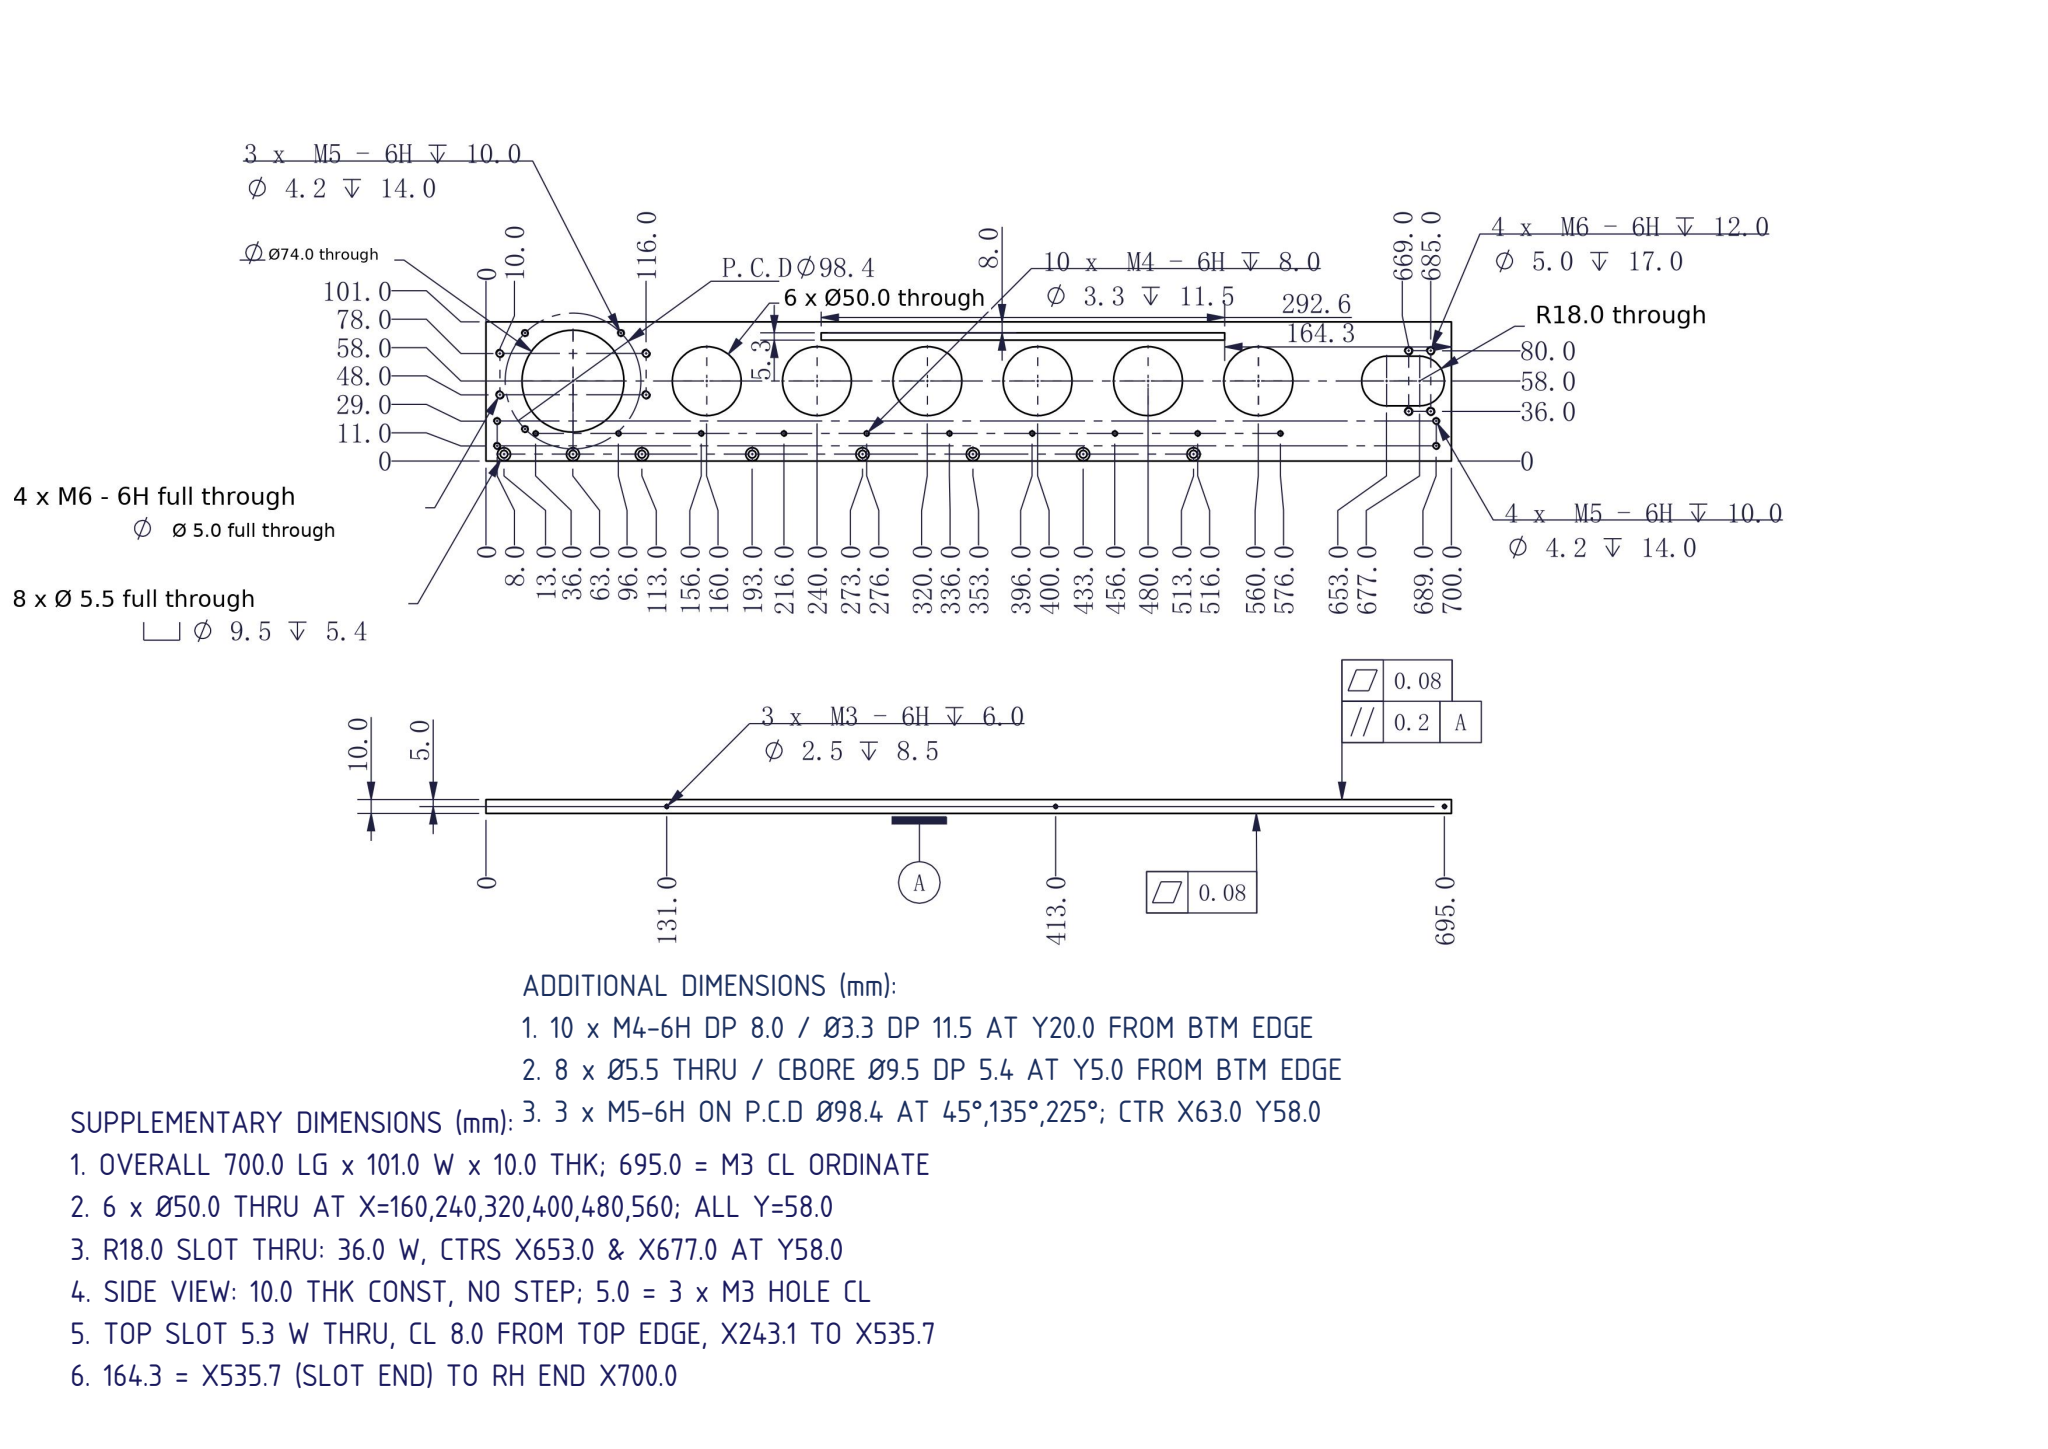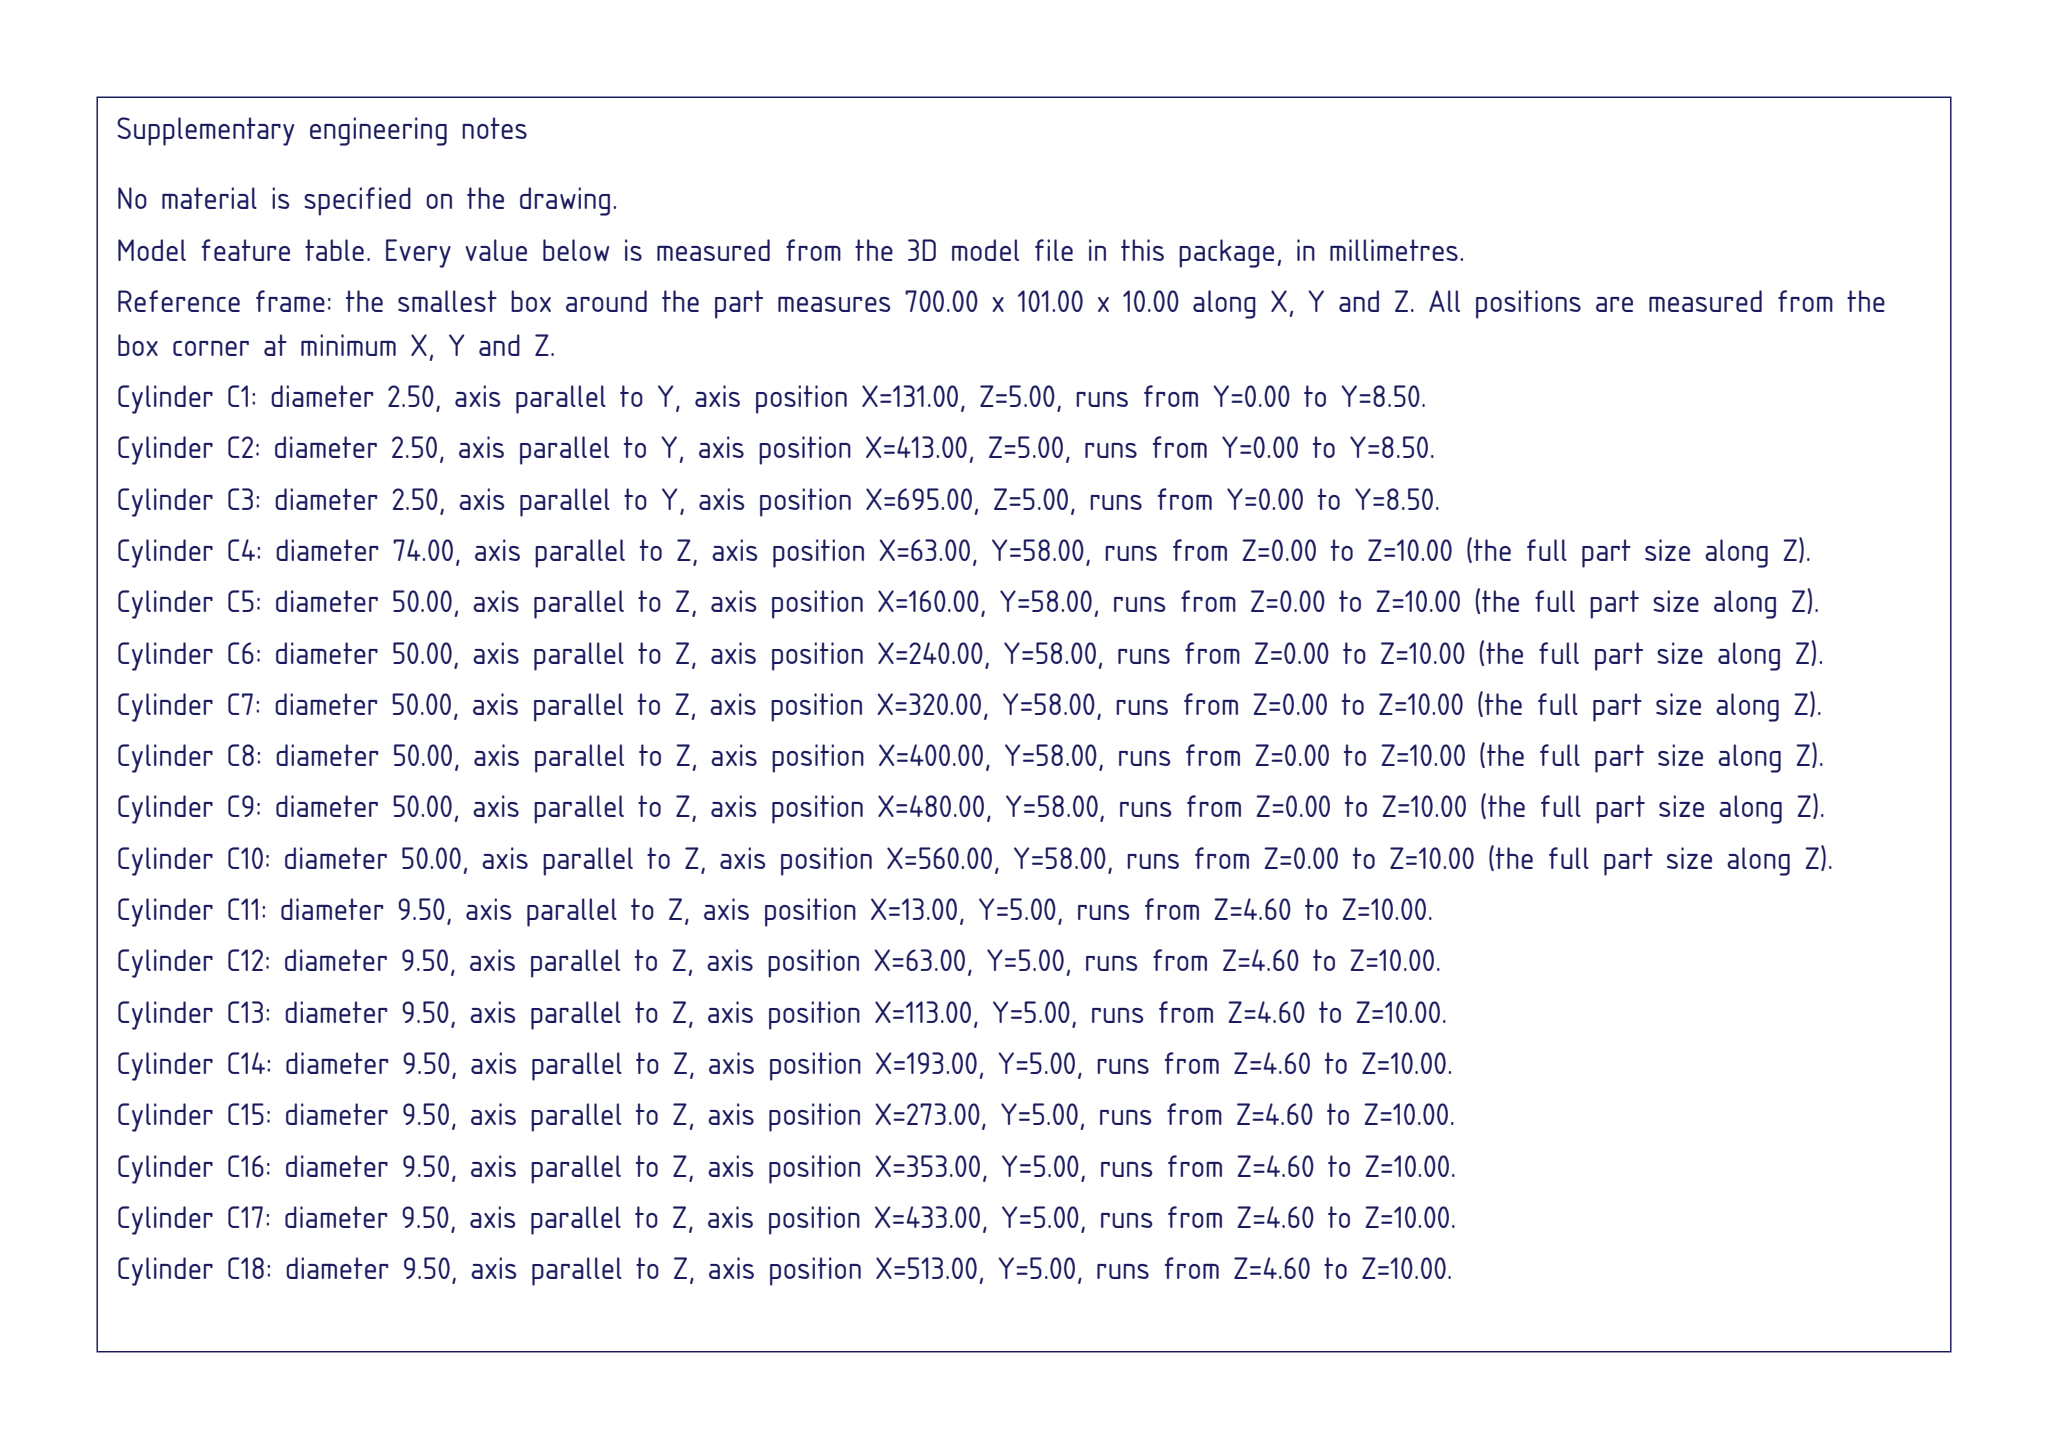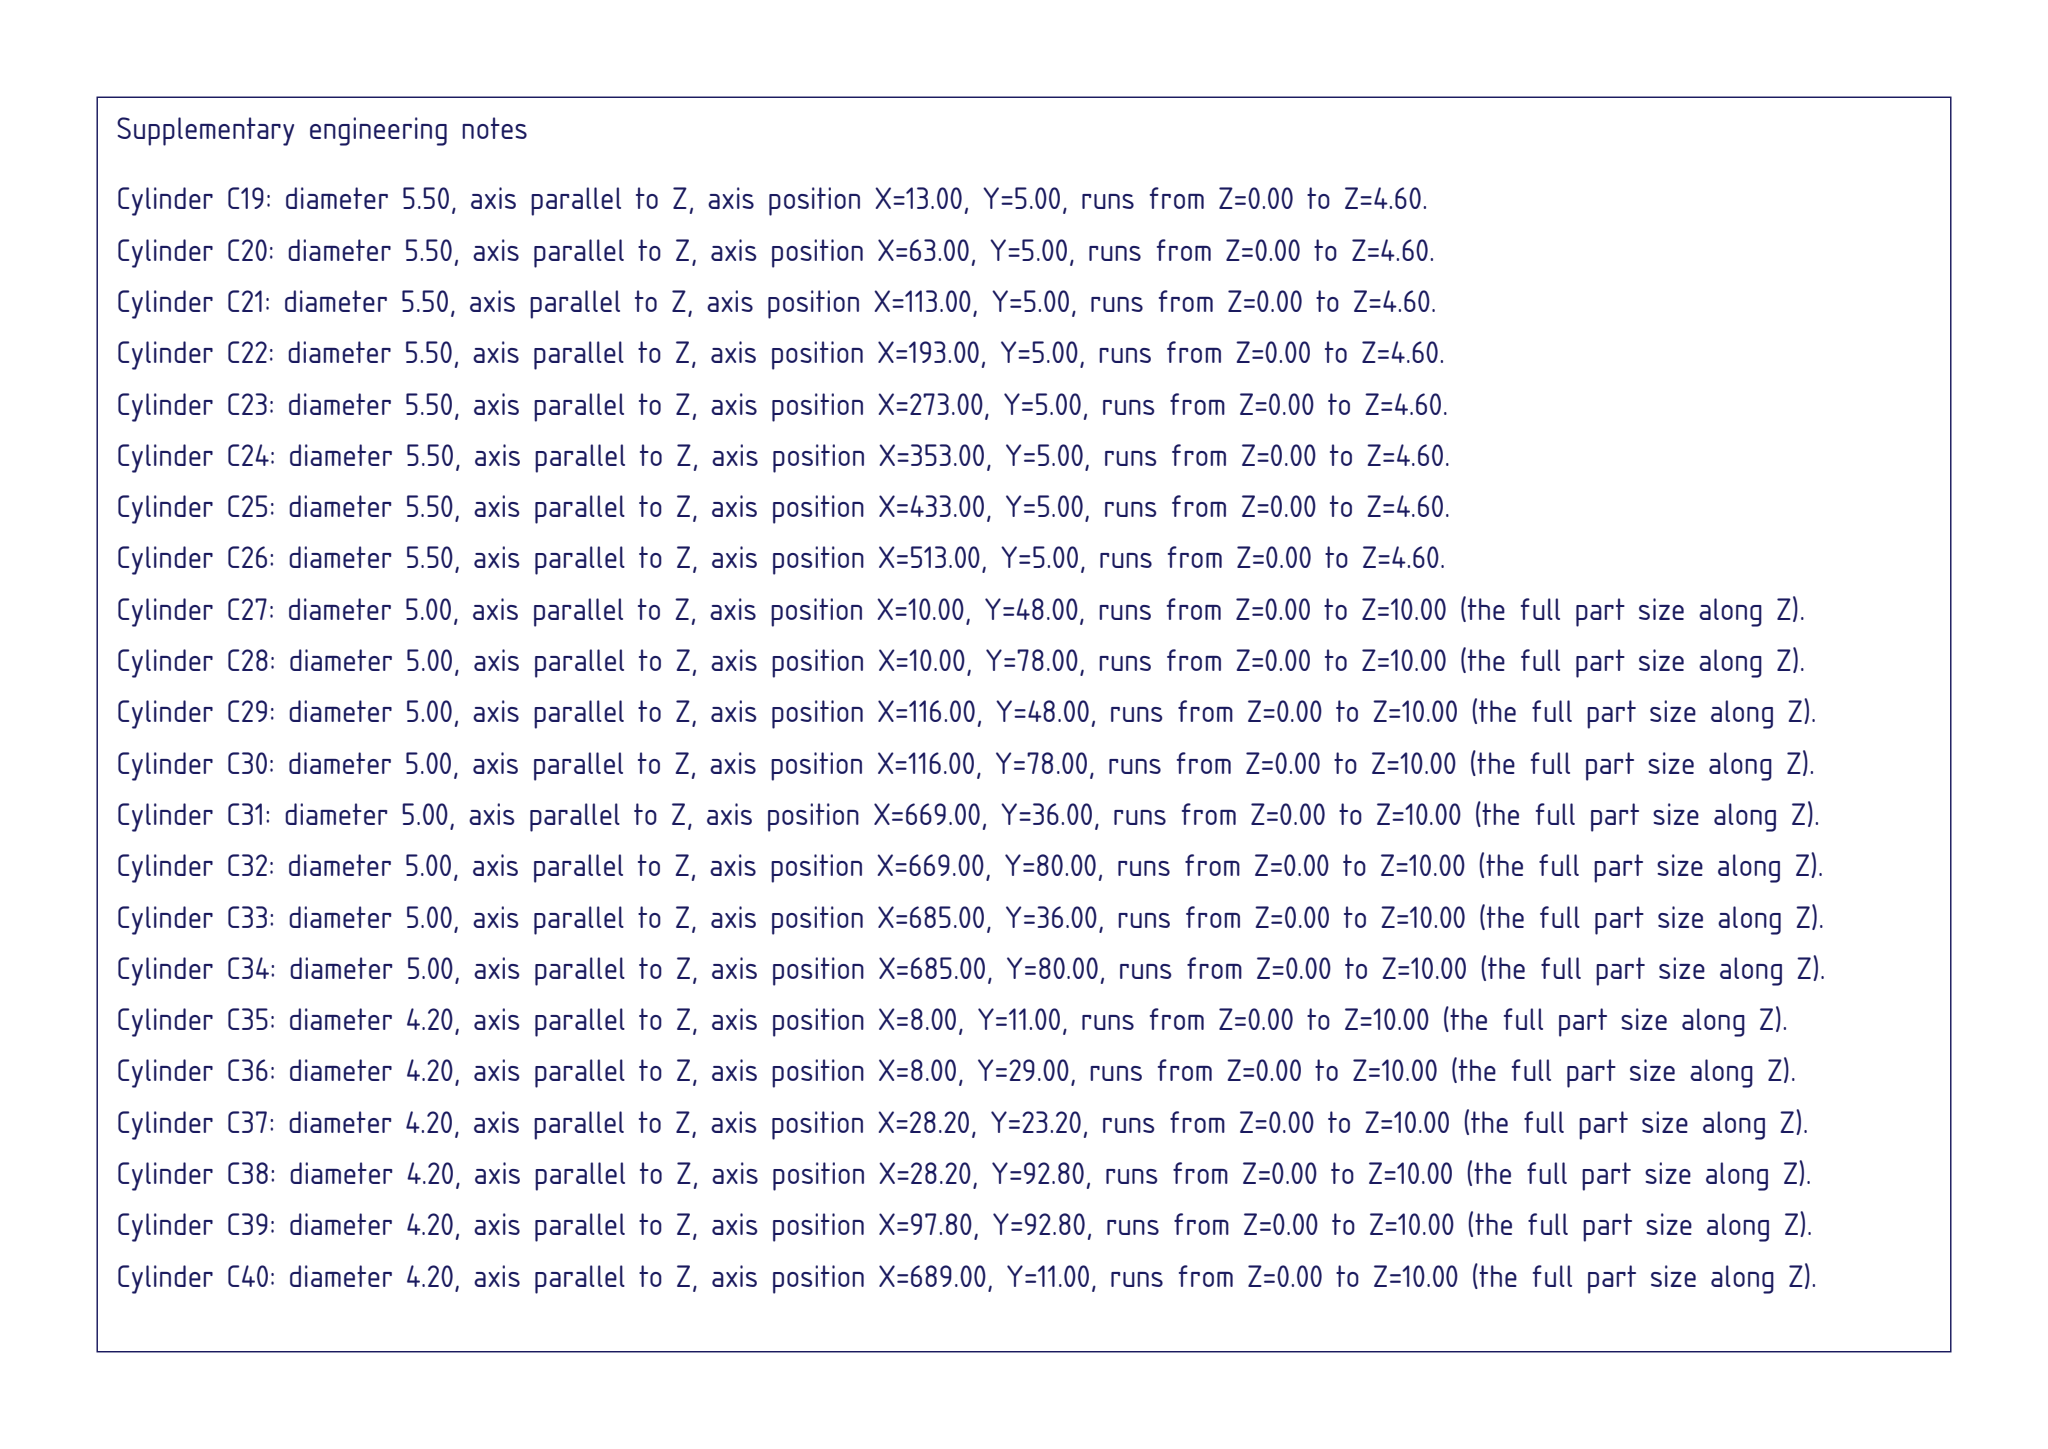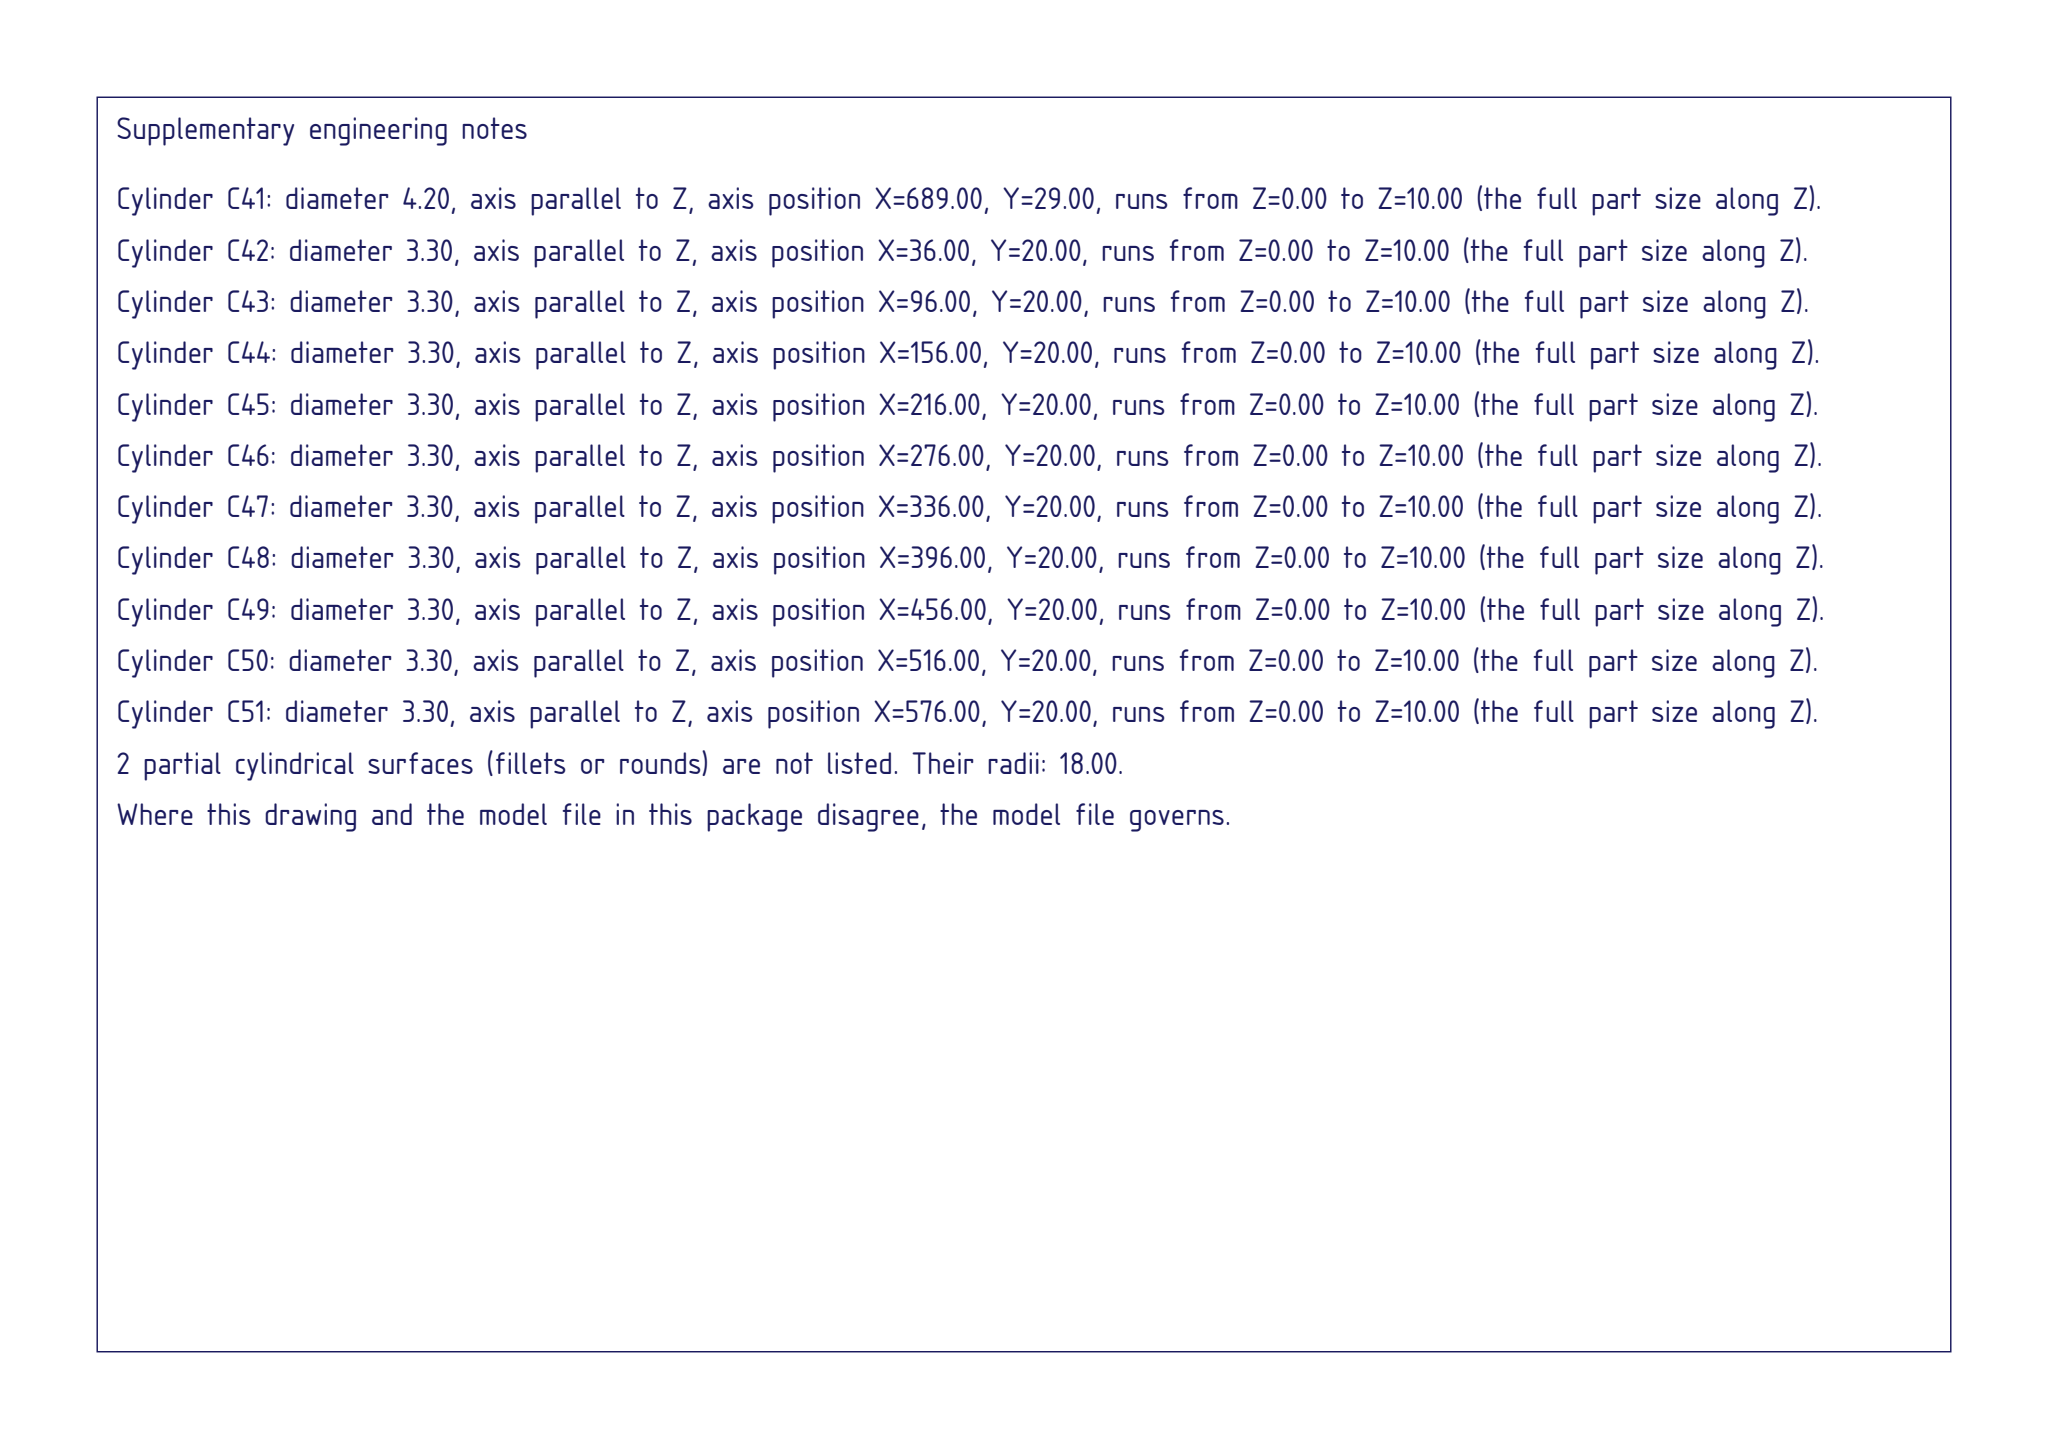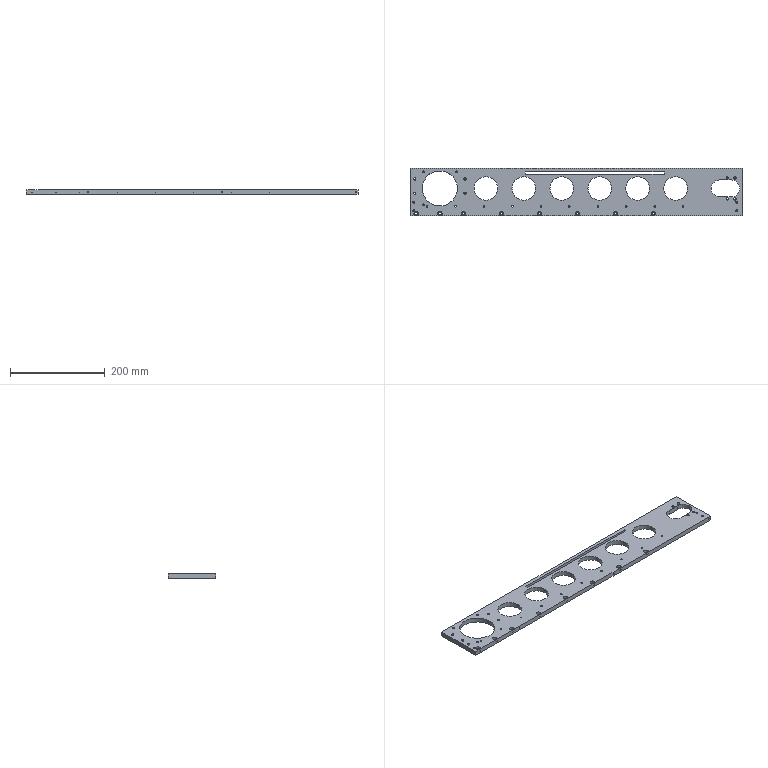Part | SolidWorks | mm | 1 solid | 131 faces | box 700 x 101 x 10 mm | volume 504520 mm3 | cylinder 105 | plane 20 | cone 6 | commonest cylinder face diameters 3.3 x20 9.5 x16 5.5 x16 5 x16 4.2 x14 50 x12 2.5 x6 36 x3
build123d program:
from build123d import *

# Parameters (mm, degrees)
SKETCH1_W                                       = 700
SKETCH1_H                                       = 116
BOSS_EXTRUDE1_DEPTH                             = 10
SKETCH2_R                                       = 37
SKETCH2_R_2                                     = 18
CUT_EXTRUDE1_DEPTH                              = 355.914
CUT_EXTRUDE3_DEPTH                              = 355.914
M5_HEX_SOCKET_HEAD_CAP_SCREW_CBORE1_D           = 5.5
M5_HEX_SOCKET_HEAD_CAP_SCREW_CBORE1_CBORE_D     = 9.5
M5_HEX_SOCKET_HEAD_CAP_SCREW_CBORE1_CBORE_DEPTH = 5.4
M3_TAPPED_HOLE1_D                               = 2.5
M3_TAPPED_HOLE1_DEPTH                           = 8.5
M3_TAPPED_HOLE1_TIP                             = 0.7511
M5_TAPPED_HOLE1_D                               = 4.2
M5_TAPPED_HOLE1_DEPTH                           = 14
M5_TAPPED_HOLE1_TIP                             = 1.262
M6_TAPPED_HOLE1_D                               = 5
M6_TAPPED_HOLE1_DEPTH                           = 17
M6_TAPPED_HOLE1_TIP                             = 1.502
M6_TAPPED_HOLE2_D                               = 5
LPATTERN1_COUNT                                 = 10
LPATTERN1_PITCH                                 = 60
CIRPATTERN1_COUNT                               = 4
SKETCH19_W                                      = 700
SKETCH19_H                                      = 15
CUT_EXTRUDE4_DEPTH                              = 355.914
SKETCH20_R                                      = 25
CUT_EXTRUDE5_DEPTH                              = 355.914
LPATTERN2_COUNT                                 = 6
LPATTERN2_PITCH                                 = 80
M5_HEX_SOCKET_HEAD_CAP_SCREW_CBORE2_D           = 5.5
M5_HEX_SOCKET_HEAD_CAP_SCREW_CBORE2_CBORE_D     = 9.5
M5_HEX_SOCKET_HEAD_CAP_SCREW_CBORE2_CBORE_DEPTH = 5.4
LPATTERN3_COUNT                                 = 5
LPATTERN3_PITCH                                 = 80
SKETCH23_W                                      = 292.572
SKETCH23_H                                      = 5.257
CUT_EXTRUDE6_DEPTH                              = 75


with BuildPart() as part:
    # Sketch1 → Boss-Extrude1 (new body)
    with BuildSketch(Plane.XY):
        Rectangle(SKETCH1_W, SKETCH1_H)
    extrude(amount=BOSS_EXTRUDE1_DEPTH)

    # Sketch2 → Cut-Extrude1 (cut, through all)
    with BuildSketch(Plane(origin=(0, 0, 0), x_dir=(-1, 0, 0), z_dir=(0, 0, -1))):
        with Locations((287, 0)):
            Circle(SKETCH2_R)
        with Locations((-315, 0)):
            Circle(SKETCH2_R_2)
    extrude(amount=-CUT_EXTRUDE1_DEPTH, mode=Mode.SUBTRACT)

    # Sketch4 → Cut-Extrude3 (cut, through all)
    with BuildSketch(Plane.XY.offset(10)):
        with BuildLine():
            Line((303, 18), (327, 18))
            ThreePointArc((327, 18), (345, 0), (327, -18))
            Line((327, -18), (303, -18))
            ThreePointArc((303, -18), (285, 0), (303, 18))
        make_face()
    extrude(amount=-CUT_EXTRUDE3_DEPTH, mode=Mode.SUBTRACT)

    # M5 Hex Socket Head Cap Screw CBORE1 (through all)
    with Locations(Plane.XY.offset(10)):
        with Locations((-237, -53), (-287, -53), (-337, -53)):
            CounterBoreHole(M5_HEX_SOCKET_HEAD_CAP_SCREW_CBORE1_D / 2, M5_HEX_SOCKET_HEAD_CAP_SCREW_CBORE1_CBORE_D / 2, M5_HEX_SOCKET_HEAD_CAP_SCREW_CBORE1_CBORE_DEPTH)

    # M3 Tapped Hole1
    with Locations(Plane(origin=(0, -58, 0), x_dir=(-1, 0, 0), z_dir=(0, -1, 0))):
        with Locations((219, -5), (-63, -5), (-345, -5)):
            Hole(M3_TAPPED_HOLE1_D / 2, depth=M3_TAPPED_HOLE1_DEPTH)
            with Locations((0, 0, -(M3_TAPPED_HOLE1_DEPTH + M3_TAPPED_HOLE1_TIP / 2))):  # 118° drill point
                Cone(0, M3_TAPPED_HOLE1_D / 2, M3_TAPPED_HOLE1_TIP, mode=Mode.SUBTRACT)

    # Sketch9 → M4 Tapped Hole1 (revolve, cut)
    with BuildSketch(Plane(origin=(-314, -38, 10), x_dir=(0, -1, 0), z_dir=(1, 0, 0))):
        Polygon((0, 0), (0, 12.491), (1.65, 11.5), (1.65, 0), align=None)
    m4_tapped_hole1 = revolve(axis=Axis((-314, -38, 16.35), (0, 0, -1)), mode=Mode.SUBTRACT)

    # M5 Tapped Hole1
    with Locations(Plane.XY.offset(10)):
        with Locations((-342, -47), (-342, -29), (339, -47), (339, -29)):
            Hole(M5_TAPPED_HOLE1_D / 2, depth=M5_TAPPED_HOLE1_DEPTH)
            with Locations((0, 0, -(M5_TAPPED_HOLE1_DEPTH + M5_TAPPED_HOLE1_TIP / 2))):  # 118° drill point
                Cone(0, M5_TAPPED_HOLE1_D / 2, M5_TAPPED_HOLE1_TIP, mode=Mode.SUBTRACT)

    # M6 Tapped Hole1
    with Locations(Plane.XY.offset(10)):
        with Locations((319, -22), (335, -22), (319, 22), (335, 22)):
            Hole(M6_TAPPED_HOLE1_D / 2, depth=M6_TAPPED_HOLE1_DEPTH)
            with Locations((0, 0, -(M6_TAPPED_HOLE1_DEPTH + M6_TAPPED_HOLE1_TIP / 2))):  # 118° drill point
                Cone(0, M6_TAPPED_HOLE1_D / 2, M6_TAPPED_HOLE1_TIP, mode=Mode.SUBTRACT)

    # Sketch15 → M5 Tapped Hole2 (revolve, cut)
    with BuildSketch(Plane(origin=(-321.8, -34.8, 10), x_dir=(0, -1, 0), z_dir=(1, 0, 0))):
        Polygon((0, 0), (0, 15.262), (2.1, 14), (2.1, 0), align=None)
    m5_tapped_hole2 = revolve(axis=Axis((-321.8, -34.8, 16.35), (0, 0, -1)), mode=Mode.SUBTRACT)

    # M6 Tapped Hole2 (through all)
    with Locations(Plane(origin=(0, 0, 0), x_dir=(-1, 0, 0), z_dir=(0, 0, -1))):
        with Locations((234, -10), (340, 20), (340, -10), (234, 20)):
            Hole(M6_TAPPED_HOLE2_D / 2)

    # LPattern1: M4 Tapped Hole1 ×10
    with Locations(*[(i * LPATTERN1_PITCH, 0, 0) for i in range(1, LPATTERN1_COUNT)]):
        add(m4_tapped_hole1, mode=Mode.SUBTRACT)

    # CirPattern1: M5 Tapped Hole2 ×4 about axis, 1 skipped
    cirpattern1_axis = Axis((-287, 0, 0), (0, 0, -1))
    add([m5_tapped_hole2.rotate(cirpattern1_axis, i * 360 / CIRPATTERN1_COUNT) for i in range(1, CIRPATTERN1_COUNT) if i not in (3,)], mode=Mode.SUBTRACT)

    # Sketch19 → Cut-Extrude4 (cut, through all)
    with BuildSketch(Plane(origin=(0, 0, 0), x_dir=(-1, 0, 0), z_dir=(0, 0, -1))):
        with Locations((0, 50.5)):
            Rectangle(SKETCH19_W, SKETCH19_H)
    extrude(amount=-CUT_EXTRUDE4_DEPTH, mode=Mode.SUBTRACT)

    # Sketch20 → Cut-Extrude5 (cut, through all)
    with BuildSketch(Plane(origin=(0, 0, 0), x_dir=(-1, 0, 0), z_dir=(0, 0, -1))):
        with Locations((-210, 0)):
            Circle(SKETCH20_R)
    cut_extrude5 = extrude(amount=-CUT_EXTRUDE5_DEPTH, mode=Mode.SUBTRACT)

    # LPattern2: Cut-Extrude5 ×6
    with Locations(*[(-i * LPATTERN2_PITCH, 0, 0) for i in range(1, LPATTERN2_COUNT)]):
        add(cut_extrude5, mode=Mode.SUBTRACT)

    # M5 Hex Socket Head Cap Screw CBORE2 (through all)
    with Locations(Plane.XY.offset(10)):
        with Locations((-157, -53)):
            m5_hex_socket_head_cap_screw_cbore2 = CounterBoreHole(M5_HEX_SOCKET_HEAD_CAP_SCREW_CBORE2_D / 2, M5_HEX_SOCKET_HEAD_CAP_SCREW_CBORE2_CBORE_D / 2, M5_HEX_SOCKET_HEAD_CAP_SCREW_CBORE2_CBORE_DEPTH)

    # LPattern3: M5 Hex Socket Head Cap Screw CBORE2 ×5
    with Locations(*[(i * LPATTERN3_PITCH, 0, 0) for i in range(1, LPATTERN3_COUNT)]):
        add(m5_hex_socket_head_cap_screw_cbore2, mode=Mode.SUBTRACT)

    # Sketch23 → Cut-Extrude6 (cut)
    with BuildSketch(Plane(origin=(0, 0, 0), x_dir=(-1, 0, 0), z_dir=(0, 0, -1))):
        with Locations((-39.393, 32.374)):
            Rectangle(SKETCH23_W, SKETCH23_H)
    extrude(amount=-CUT_EXTRUDE6_DEPTH, mode=Mode.SUBTRACT)


solid = part.part